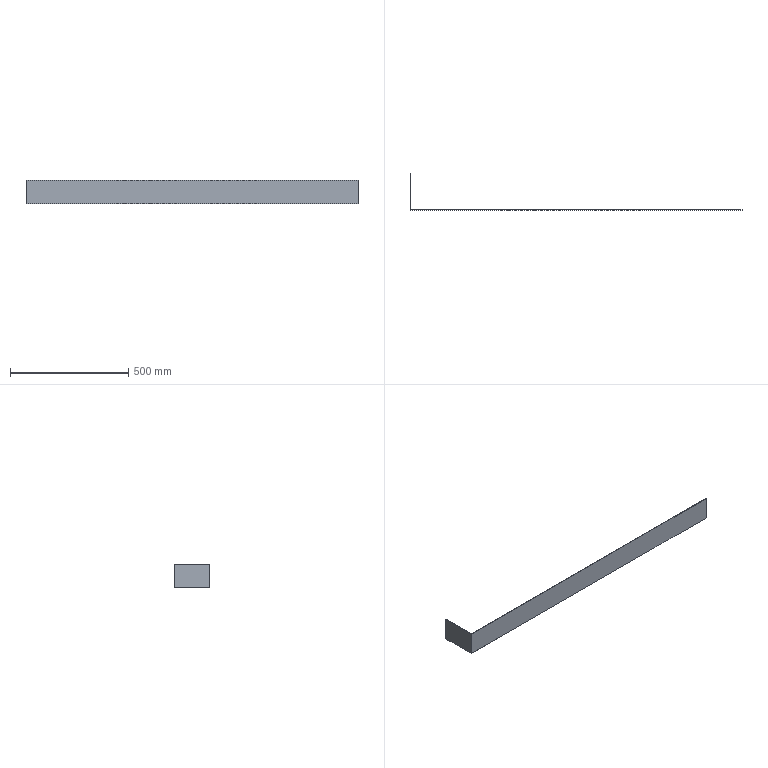Component | SolidWorks | LD101-02-Product-Q1-2-3-2 | 1 solid | 8 faces | box 1402 x 152 x 100 mm | volume 310400 mm3 | plane 8 | material POM (White)
build123d program:
from build123d import *

# Parameters (mm, degrees)
EXTRUDE_THIN1_DEPTH = 50


with BuildPart() as part:
    # Sketch1 → Extrude-Thin1 (new, symmetric)
    with BuildSketch(Plane.XY):
        Polygon((0, 150), (0, 0), (1400, 0), (1400, -2), (-2, -2), (-2, 150), align=None)
    extrude(amount=EXTRUDE_THIN1_DEPTH, both=True)


solid = part.part

# Placed as in the assembly
solid = solid.moved(Location((-970.29, -146.897, 217.257), (0, 0, 0)))
STEP:
#1=CARTESIAN_POINT('',(-38.279,-5.862,6.585));
#2=VERTEX_POINT('',#1);
#3=CARTESIAN_POINT('',(16.918,-5.862,6.585));
#4=VERTEX_POINT('',#3);
#5=CARTESIAN_POINT('',(-38.2,-5.862,6.585));
#6=DIRECTION('',(1.,0.,0.));
#7=VECTOR('',#6,39.37);
#8=LINE('',#5,#7);
#9=EDGE_CURVE('',#2,#4,#8,.T.);
#10=ORIENTED_EDGE('',*,*,#9,.T.);
#11=CARTESIAN_POINT('',(16.918,-5.862,10.522));
#12=VERTEX_POINT('',#11);
#13=CARTESIAN_POINT('',(16.918,-5.862,10.522));
#14=DIRECTION('',(0.,0.,-1.));
#15=VECTOR('',#14,39.37);
#16=LINE('',#13,#15);
#17=EDGE_CURVE('',#12,#4,#16,.T.);
#18=ORIENTED_EDGE('',*,*,#17,.F.);
#19=CARTESIAN_POINT('',(-38.279,-5.862,10.522));
#20=VERTEX_POINT('',#19);
#21=CARTESIAN_POINT('',(-38.2,-5.862,10.522));
#22=DIRECTION('',(1.,0.,0.));
#23=VECTOR('',#22,39.37);
#24=LINE('',#21,#23);
#25=EDGE_CURVE('',#20,#12,#24,.T.);
#26=ORIENTED_EDGE('',*,*,#25,.F.);
#27=CARTESIAN_POINT('',(-38.279,-5.862,10.522));
#28=DIRECTION('',(0.,0.,-1.));
#29=VECTOR('',#28,39.37);
#30=LINE('',#27,#29);
#31=EDGE_CURVE('',#20,#2,#30,.T.);
#32=ORIENTED_EDGE('',*,*,#31,.T.);
#33=EDGE_LOOP('',(#10,#18,#26,#32));
#34=FACE_OUTER_BOUND('',#33,.T.);
#35=CARTESIAN_POINT('',(-38.2,-5.862,10.522));
#36=DIRECTION('',(0.,1.,0.));
#37=DIRECTION('',(0.,0.,1.));
#38=AXIS2_PLACEMENT_3D('',#35,#36,#37);
#39=PLANE('',#38);
#40=ADVANCED_FACE('',(#34),#39,.F.);
#41=CARTESIAN_POINT('',(16.918,-5.783,6.585));
#42=VERTEX_POINT('',#41);
#43=CARTESIAN_POINT('',(16.918,-5.783,6.585));
#44=DIRECTION('',(0.,-1.,0.));
#45=VECTOR('',#44,39.37);
#46=LINE('',#43,#45);
#47=EDGE_CURVE('',#42,#4,#46,.T.);
#48=ORIENTED_EDGE('',*,*,#47,.F.);
#49=CARTESIAN_POINT('',(16.918,-5.783,10.522));
#50=VERTEX_POINT('',#49);
#51=CARTESIAN_POINT('',(16.918,-5.783,10.522));
#52=DIRECTION('',(0.,0.,-1.));
#53=VECTOR('',#52,39.37);
#54=LINE('',#51,#53);
#55=EDGE_CURVE('',#50,#42,#54,.T.);
#56=ORIENTED_EDGE('',*,*,#55,.F.);
#57=CARTESIAN_POINT('',(16.918,-5.783,10.522));
#58=DIRECTION('',(0.,-1.,0.));
#59=VECTOR('',#58,39.37);
#60=LINE('',#57,#59);
#61=EDGE_CURVE('',#50,#12,#60,.T.);
#62=ORIENTED_EDGE('',*,*,#61,.T.);
#63=ORIENTED_EDGE('',*,*,#17,.T.);
#64=EDGE_LOOP('',(#48,#56,#62,#63));
#65=FACE_OUTER_BOUND('',#64,.T.);
#66=CARTESIAN_POINT('',(16.918,-5.783,10.522));
#67=DIRECTION('',(1.,0.,0.));
#68=DIRECTION('',(0.,0.,-1.));
#69=AXIS2_PLACEMENT_3D('',#66,#67,#68);
#70=PLANE('',#69);
#71=ADVANCED_FACE('',(#65),#70,.T.);
#72=CARTESIAN_POINT('',(-38.2,-5.783,6.585));
#73=VERTEX_POINT('',#72);
#74=CARTESIAN_POINT('',(-38.2,-5.783,6.585));
#75=DIRECTION('',(1.,0.,0.));
#76=VECTOR('',#75,39.37);
#77=LINE('',#74,#76);
#78=EDGE_CURVE('',#73,#42,#77,.T.);
#79=ORIENTED_EDGE('',*,*,#78,.F.);
#80=CARTESIAN_POINT('',(-38.2,-5.783,10.522));
#81=VERTEX_POINT('',#80);
#82=CARTESIAN_POINT('',(-38.2,-5.783,10.522));
#83=DIRECTION('',(0.,0.,-1.));
#84=VECTOR('',#83,39.37);
#85=LINE('',#82,#84);
#86=EDGE_CURVE('',#81,#73,#85,.T.);
#87=ORIENTED_EDGE('',*,*,#86,.F.);
#88=CARTESIAN_POINT('',(-38.2,-5.783,10.522));
#89=DIRECTION('',(1.,0.,0.));
#90=VECTOR('',#89,39.37);
#91=LINE('',#88,#90);
#92=EDGE_CURVE('',#81,#50,#91,.T.);
#93=ORIENTED_EDGE('',*,*,#92,.T.);
#94=ORIENTED_EDGE('',*,*,#55,.T.);
#95=EDGE_LOOP('',(#79,#87,#93,#94));
#96=FACE_OUTER_BOUND('',#95,.T.);
#97=CARTESIAN_POINT('',(-38.2,-5.783,10.522));
#98=DIRECTION('',(0.,1.,0.));
#99=DIRECTION('',(0.,0.,1.));
#100=AXIS2_PLACEMENT_3D('',#97,#98,#99);
#101=PLANE('',#100);
#102=ADVANCED_FACE('',(#96),#101,.T.);
#103=CARTESIAN_POINT('',(-38.2,0.1222,6.585));
#104=VERTEX_POINT('',#103);
#105=CARTESIAN_POINT('',(-38.2,0.1222,6.585));
#106=DIRECTION('',(0.,-1.,0.));
#107=VECTOR('',#106,39.37);
#108=LINE('',#105,#107);
#109=EDGE_CURVE('',#104,#73,#108,.T.);
#110=ORIENTED_EDGE('',*,*,#109,.F.);
#111=CARTESIAN_POINT('',(-38.2,0.1222,10.522));
#112=VERTEX_POINT('',#111);
#113=CARTESIAN_POINT('',(-38.2,0.1222,10.522));
#114=DIRECTION('',(0.,0.,-1.));
#115=VECTOR('',#114,39.37);
#116=LINE('',#113,#115);
#117=EDGE_CURVE('',#112,#104,#116,.T.);
#118=ORIENTED_EDGE('',*,*,#117,.F.);
#119=CARTESIAN_POINT('',(-38.2,0.1222,10.522));
#120=DIRECTION('',(0.,-1.,0.));
#121=VECTOR('',#120,39.37);
#122=LINE('',#119,#121);
#123=EDGE_CURVE('',#112,#81,#122,.T.);
#124=ORIENTED_EDGE('',*,*,#123,.T.);
#125=ORIENTED_EDGE('',*,*,#86,.T.);
#126=EDGE_LOOP('',(#110,#118,#124,#125));
#127=FACE_OUTER_BOUND('',#126,.T.);
#128=CARTESIAN_POINT('',(-38.2,0.1222,10.522));
#129=DIRECTION('',(1.,0.,0.));
#130=DIRECTION('',(-0.,1.,0.));
#131=AXIS2_PLACEMENT_3D('',#128,#129,#130);
#132=PLANE('',#131);
#133=ADVANCED_FACE('',(#127),#132,.T.);
#134=CARTESIAN_POINT('',(-38.279,0.1222,6.585));
#135=VERTEX_POINT('',#134);
#136=CARTESIAN_POINT('',(-38.279,0.1222,6.585));
#137=DIRECTION('',(1.,0.,0.));
#138=VECTOR('',#137,39.37);
#139=LINE('',#136,#138);
#140=EDGE_CURVE('',#135,#104,#139,.T.);
#141=ORIENTED_EDGE('',*,*,#140,.F.);
#142=CARTESIAN_POINT('',(-38.279,0.1222,10.522));
#143=VERTEX_POINT('',#142);
#144=CARTESIAN_POINT('',(-38.279,0.1222,10.522));
#145=DIRECTION('',(0.,0.,-1.));
#146=VECTOR('',#145,39.37);
#147=LINE('',#144,#146);
#148=EDGE_CURVE('',#143,#135,#147,.T.);
#149=ORIENTED_EDGE('',*,*,#148,.F.);
#150=CARTESIAN_POINT('',(-38.279,0.1222,10.522));
#151=DIRECTION('',(1.,0.,0.));
#152=VECTOR('',#151,39.37);
#153=LINE('',#150,#152);
#154=EDGE_CURVE('',#143,#112,#153,.T.);
#155=ORIENTED_EDGE('',*,*,#154,.T.);
#156=ORIENTED_EDGE('',*,*,#117,.T.);
#157=EDGE_LOOP('',(#141,#149,#155,#156));
#158=FACE_OUTER_BOUND('',#157,.T.);
#159=CARTESIAN_POINT('',(-38.279,0.1222,10.522));
#160=DIRECTION('',(0.,1.,0.));
#161=DIRECTION('',(0.,0.,1.));
#162=AXIS2_PLACEMENT_3D('',#159,#160,#161);
#163=PLANE('',#162);
#164=ADVANCED_FACE('',(#158),#163,.T.);
#165=CARTESIAN_POINT('',(-38.279,0.1222,6.585));
#166=DIRECTION('',(0.,-1.,0.));
#167=VECTOR('',#166,39.37);
#168=LINE('',#165,#167);
#169=EDGE_CURVE('',#135,#2,#168,.T.);
#170=ORIENTED_EDGE('',*,*,#169,.T.);
#171=ORIENTED_EDGE('',*,*,#31,.F.);
#172=CARTESIAN_POINT('',(-38.279,0.1222,10.522));
#173=DIRECTION('',(0.,-1.,0.));
#174=VECTOR('',#173,39.37);
#175=LINE('',#172,#174);
#176=EDGE_CURVE('',#143,#20,#175,.T.);
#177=ORIENTED_EDGE('',*,*,#176,.F.);
#178=ORIENTED_EDGE('',*,*,#148,.T.);
#179=EDGE_LOOP('',(#170,#171,#177,#178));
#180=FACE_OUTER_BOUND('',#179,.T.);
#181=CARTESIAN_POINT('',(-38.279,0.1222,10.522));
#182=DIRECTION('',(1.,0.,0.));
#183=DIRECTION('',(-0.,1.,0.));
#184=AXIS2_PLACEMENT_3D('',#181,#182,#183);
#185=PLANE('',#184);
#186=ADVANCED_FACE('',(#180),#185,.F.);
#187=ORIENTED_EDGE('',*,*,#25,.T.);
#188=ORIENTED_EDGE('',*,*,#61,.F.);
#189=ORIENTED_EDGE('',*,*,#92,.F.);
#190=ORIENTED_EDGE('',*,*,#123,.F.);
#191=ORIENTED_EDGE('',*,*,#154,.F.);
#192=ORIENTED_EDGE('',*,*,#176,.T.);
#193=EDGE_LOOP('',(#187,#188,#189,#190,#191,#192));
#194=FACE_OUTER_BOUND('',#193,.T.);
#195=CARTESIAN_POINT('',(-38.2,-5.783,10.522));
#196=DIRECTION('',(0.,0.,-1.));
#197=DIRECTION('',(-1.,0.,0.));
#198=AXIS2_PLACEMENT_3D('',#195,#196,#197);
#199=PLANE('',#198);
#200=ADVANCED_FACE('',(#194),#199,.F.);
#201=ORIENTED_EDGE('',*,*,#9,.F.);
#202=ORIENTED_EDGE('',*,*,#169,.F.);
#203=ORIENTED_EDGE('',*,*,#140,.T.);
#204=ORIENTED_EDGE('',*,*,#109,.T.);
#205=ORIENTED_EDGE('',*,*,#78,.T.);
#206=ORIENTED_EDGE('',*,*,#47,.T.);
#207=EDGE_LOOP('',(#201,#202,#203,#204,#205,#206));
#208=FACE_OUTER_BOUND('',#207,.T.);
#209=CARTESIAN_POINT('',(-38.2,-5.783,6.585));
#210=DIRECTION('',(0.,0.,-1.));
#211=DIRECTION('',(-1.,0.,0.));
#212=AXIS2_PLACEMENT_3D('',#209,#210,#211);
#213=PLANE('',#212);
#214=ADVANCED_FACE('',(#208),#213,.T.);
#215=CLOSED_SHELL('',(#40,#71,#102,#133,#164,#186,#200,#214));
#216=MANIFOLD_SOLID_BREP('',#215);
#217=CARTESIAN_POINT('',(0.,0.,0.));
#218=DIRECTION('',(0.,0.,1.));
#219=DIRECTION('',(1.,0.,0.));
#220=AXIS2_PLACEMENT_3D('',#217,#218,#219);
#221=(LENGTH_UNIT()NAMED_UNIT(*)SI_UNIT($,.METRE.));
#222=LENGTH_MEASURE_WITH_UNIT(LENGTH_MEASURE(0.0254),#221);
#223=DIMENSIONAL_EXPONENTS(1.,0.,0.,0.,0.,0.,0.);
#224=(CONVERSION_BASED_UNIT('',#222)LENGTH_UNIT()NAMED_UNIT(#223));
#225=UNCERTAINTY_MEASURE_WITH_UNIT(LENGTH_MEASURE(0.00001),#224,'','');
#226=(NAMED_UNIT(*)PLANE_ANGLE_UNIT()SI_UNIT($,.RADIAN.));
#227=(NAMED_UNIT(*)SI_UNIT($,.STERADIAN.)SOLID_ANGLE_UNIT());
#228=(GEOMETRIC_REPRESENTATION_CONTEXT(3)GLOBAL_UNCERTAINTY_ASSIGNED_CONTEXT((#225))GLOBAL_UNIT_ASSIGNED_CONTEXT((#224,#226,#227))REPRESENTATION_CONTEXT('',''));
#229=ADVANCED_BREP_SHAPE_REPRESENTATION('',(#216,#220),#228);
#230=COLOUR_RGB('',0.7922,0.8196,0.9333);
#231=FILL_AREA_STYLE_COLOUR('',#230);
#232=FILL_AREA_STYLE('',(#231));
#233=SURFACE_STYLE_FILL_AREA(#232);
#234=SURFACE_SIDE_STYLE('',(#233));
#235=SURFACE_STYLE_USAGE(.BOTH.,#234);
#236=PRESENTATION_STYLE_ASSIGNMENT((#235));
#237=STYLED_ITEM('',(#236),#216);
#238=PRESENTATION_LAYER_ASSIGNMENT('','',(#237));
#239=(LENGTH_UNIT()NAMED_UNIT(*)SI_UNIT($,.METRE.));
#240=LENGTH_MEASURE_WITH_UNIT(LENGTH_MEASURE(0.0254),#239);
#241=DIMENSIONAL_EXPONENTS(1.,0.,0.,0.,0.,0.,0.);
#242=(CONVERSION_BASED_UNIT('',#240)LENGTH_UNIT()NAMED_UNIT(#241));
#243=UNCERTAINTY_MEASURE_WITH_UNIT(LENGTH_MEASURE(0.00001),#242,'','');
#244=(NAMED_UNIT(*)PLANE_ANGLE_UNIT()SI_UNIT($,.RADIAN.));
#245=(NAMED_UNIT(*)SI_UNIT($,.STERADIAN.)SOLID_ANGLE_UNIT());
#246=(GEOMETRIC_REPRESENTATION_CONTEXT(3)GLOBAL_UNCERTAINTY_ASSIGNED_CONTEXT((#243))GLOBAL_UNIT_ASSIGNED_CONTEXT((#242,#244,#245))REPRESENTATION_CONTEXT('',''));
#247=MECHANICAL_DESIGN_GEOMETRIC_PRESENTATION_REPRESENTATION('',(#237),#246);